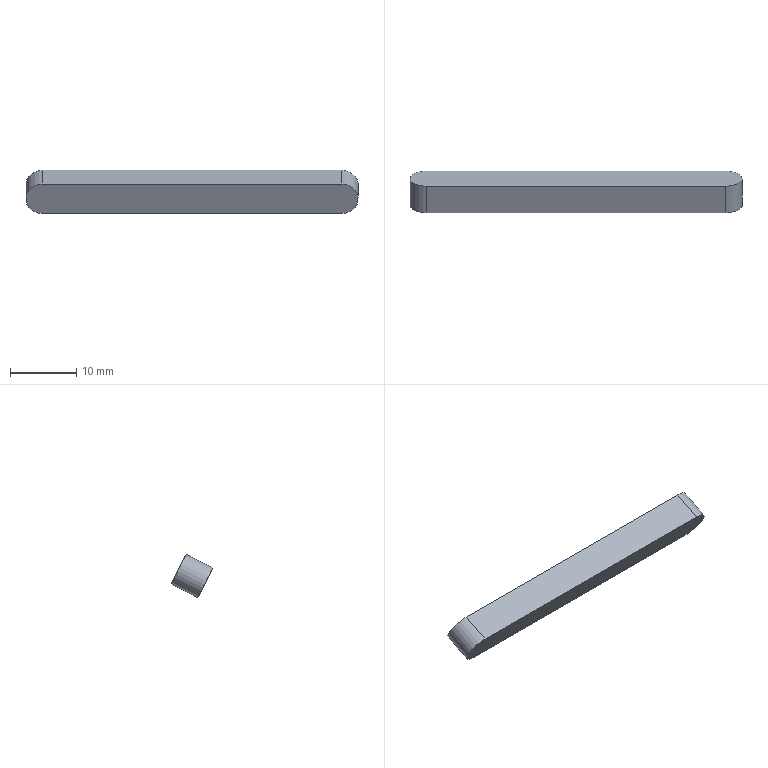Component | NX | KEY | 1 solid | 6 faces | box 50 x 6.28 x 6.5 mm | volume 1101 mm3 | plane 4 | cylinder 2 | commonest cylinder face diameters 5 x2
STEP:
#1=CARTESIAN_POINT('',(0.,0.,0.));
#2=DIRECTION('',(0.,0.,1.));
#3=DIRECTION('',(1.,0.,0.));
#4=AXIS2_PLACEMENT_3D('',#1,#2,#3);
#5=CARTESIAN_POINT('',(48.5,6.481,123.503));
#6=VERTEX_POINT('',#5);
#7=CARTESIAN_POINT('',(48.5,4.206,127.956));
#8=VERTEX_POINT('',#7);
#9=CARTESIAN_POINT('',(48.5,5.343,125.729));
#10=DIRECTION('',(0.,0.8906,0.4549));
#11=DIRECTION('',(1.,0.,0.));
#12=AXIS2_PLACEMENT_3D('',#9,#10,#11);
#13=CIRCLE('',#12,2.5);
#14=CARTESIAN_POINT('',(48.5,9.351,127.776));
#15=DIRECTION('',(0.,-0.8906,-0.4549));
#16=DIRECTION('',(-1.,0.,0.));
#17=AXIS2_PLACEMENT_3D('',#14,#15,#16);
#18=CYLINDRICAL_SURFACE('',#17,2.5);
#19=CARTESIAN_POINT('',(3.142,4.5));
#20=DIRECTION('',(-1.,-0.));
#21=VECTOR('',#20,1.);
#22=LINE('',#19,#21);
#23=(GEOMETRIC_REPRESENTATION_CONTEXT(2)PARAMETRIC_REPRESENTATION_CONTEXT()REPRESENTATION_CONTEXT('',''));
#24=DEFINITIONAL_REPRESENTATION('',(#22),#23);
#25=PCURVE('',#18,#24);
#26=CARTESIAN_POINT('',(48.5,5.343,125.729));
#27=DIRECTION('',(0.,0.8906,0.4549));
#28=DIRECTION('',(1.,0.,0.));
#29=AXIS2_PLACEMENT_3D('',#26,#27,#28);
#30=PLANE('',#29);
#31=CARTESIAN_POINT('',(0.,0.));
#32=DIRECTION('',(1.,0.));
#33=AXIS2_PLACEMENT_2D('',#31,#32);
#34=CIRCLE('',#33,2.5);
#35=(GEOMETRIC_REPRESENTATION_CONTEXT(2)PARAMETRIC_REPRESENTATION_CONTEXT()REPRESENTATION_CONTEXT('',''));
#36=DEFINITIONAL_REPRESENTATION('',(#34),#35);
#37=PCURVE('',#30,#36);
#38=SURFACE_CURVE('',#13,(#25,#37),.PCURVE_S1.);
#39=EDGE_CURVE('',#6,#8,#38,.T.);
#40=ORIENTED_EDGE('',*,*,#39,.T.);
#41=CARTESIAN_POINT('',(48.5,8.214,130.003));
#42=VERTEX_POINT('',#41);
#43=CARTESIAN_POINT('',(48.5,8.214,130.003));
#44=DIRECTION('',(0.,-0.8906,-0.4549));
#45=VECTOR('',#44,1.);
#46=LINE('',#43,#45);
#47=CARTESIAN_POINT('',(-1.571,-0.));
#48=DIRECTION('',(0.,1.));
#49=VECTOR('',#48,1.);
#50=LINE('',#47,#49);
#51=(GEOMETRIC_REPRESENTATION_CONTEXT(2)PARAMETRIC_REPRESENTATION_CONTEXT()REPRESENTATION_CONTEXT('',''));
#52=DEFINITIONAL_REPRESENTATION('',(#50),#51);
#53=PCURVE('',#18,#52);
#54=CARTESIAN_POINT('',(48.5,8.214,130.003));
#55=DIRECTION('',(0.,0.4549,-0.8906));
#56=DIRECTION('',(0.,0.8906,0.4549));
#57=AXIS2_PLACEMENT_3D('',#54,#55,#56);
#58=PLANE('',#57);
#59=CARTESIAN_POINT('',(0.,0.));
#60=DIRECTION('',(-1.,0.));
#61=VECTOR('',#60,1.);
#62=LINE('',#59,#61);
#63=(GEOMETRIC_REPRESENTATION_CONTEXT(2)PARAMETRIC_REPRESENTATION_CONTEXT()REPRESENTATION_CONTEXT('',''));
#64=DEFINITIONAL_REPRESENTATION('',(#62),#63);
#65=PCURVE('',#58,#64);
#66=SURFACE_CURVE('',#46,(#53,#65),.PCURVE_S1.);
#67=EDGE_CURVE('',#42,#8,#66,.T.);
#68=ORIENTED_EDGE('',*,*,#67,.F.);
#69=CARTESIAN_POINT('',(48.5,10.488,125.55));
#70=VERTEX_POINT('',#69);
#71=CARTESIAN_POINT('',(48.5,9.351,127.776));
#72=DIRECTION('',(0.,0.8906,0.4549));
#73=DIRECTION('',(1.,0.,0.));
#74=AXIS2_PLACEMENT_3D('',#71,#72,#73);
#75=CIRCLE('',#74,2.5);
#76=CARTESIAN_POINT('',(3.142,0.));
#77=DIRECTION('',(-1.,-0.));
#78=VECTOR('',#77,1.);
#79=LINE('',#76,#78);
#80=(GEOMETRIC_REPRESENTATION_CONTEXT(2)PARAMETRIC_REPRESENTATION_CONTEXT()REPRESENTATION_CONTEXT('',''));
#81=DEFINITIONAL_REPRESENTATION('',(#79),#80);
#82=PCURVE('',#18,#81);
#83=CARTESIAN_POINT('',(48.5,9.351,127.776));
#84=DIRECTION('',(0.,0.8906,0.4549));
#85=DIRECTION('',(1.,0.,0.));
#86=AXIS2_PLACEMENT_3D('',#83,#84,#85);
#87=PLANE('',#86);
#88=CARTESIAN_POINT('',(0.,0.));
#89=DIRECTION('',(1.,0.));
#90=AXIS2_PLACEMENT_2D('',#88,#89);
#91=CIRCLE('',#90,2.5);
#92=(GEOMETRIC_REPRESENTATION_CONTEXT(2)PARAMETRIC_REPRESENTATION_CONTEXT()REPRESENTATION_CONTEXT('',''));
#93=DEFINITIONAL_REPRESENTATION('',(#91),#92);
#94=PCURVE('',#87,#93);
#95=SURFACE_CURVE('',#75,(#82,#94),.PCURVE_S1.);
#96=EDGE_CURVE('',#70,#42,#95,.T.);
#97=ORIENTED_EDGE('',*,*,#96,.F.);
#98=CARTESIAN_POINT('',(48.5,10.488,125.55));
#99=DIRECTION('',(0.,-0.8906,-0.4549));
#100=VECTOR('',#99,1.);
#101=LINE('',#98,#100);
#102=CARTESIAN_POINT('',(1.571,0.));
#103=DIRECTION('',(0.,1.));
#104=VECTOR('',#103,1.);
#105=LINE('',#102,#104);
#106=(GEOMETRIC_REPRESENTATION_CONTEXT(2)PARAMETRIC_REPRESENTATION_CONTEXT()REPRESENTATION_CONTEXT('',''));
#107=DEFINITIONAL_REPRESENTATION('',(#105),#106);
#108=PCURVE('',#18,#107);
#109=CARTESIAN_POINT('',(93.5,10.488,125.55));
#110=DIRECTION('',(0.,-0.4549,0.8906));
#111=DIRECTION('',(0.,-0.8906,-0.4549));
#112=AXIS2_PLACEMENT_3D('',#109,#110,#111);
#113=PLANE('',#112);
#114=CARTESIAN_POINT('',(0.,-45.));
#115=DIRECTION('',(1.,0.));
#116=VECTOR('',#115,1.);
#117=LINE('',#114,#116);
#118=(GEOMETRIC_REPRESENTATION_CONTEXT(2)PARAMETRIC_REPRESENTATION_CONTEXT()REPRESENTATION_CONTEXT('',''));
#119=DEFINITIONAL_REPRESENTATION('',(#117),#118);
#120=PCURVE('',#113,#119);
#121=SURFACE_CURVE('',#101,(#108,#120),.PCURVE_S1.);
#122=EDGE_CURVE('',#70,#6,#121,.T.);
#123=ORIENTED_EDGE('',*,*,#122,.T.);
#124=EDGE_LOOP('',(#40,#68,#97,#123));
#125=FACE_BOUND('',#124,.T.);
#126=ADVANCED_FACE('',(#125),#18,.T.);
#127=CARTESIAN_POINT('',(93.5,4.206,127.956));
#128=VERTEX_POINT('',#127);
#129=CARTESIAN_POINT('',(48.5,4.206,127.956));
#130=DIRECTION('',(1.,0.,0.));
#131=VECTOR('',#130,1.);
#132=LINE('',#129,#131);
#133=CARTESIAN_POINT('',(-4.5,0.));
#134=DIRECTION('',(0.,1.));
#135=VECTOR('',#134,1.);
#136=LINE('',#133,#135);
#137=(GEOMETRIC_REPRESENTATION_CONTEXT(2)PARAMETRIC_REPRESENTATION_CONTEXT()REPRESENTATION_CONTEXT('',''));
#138=DEFINITIONAL_REPRESENTATION('',(#136),#137);
#139=PCURVE('',#58,#138);
#140=CARTESIAN_POINT('',(0.,-2.5));
#141=DIRECTION('',(1.,0.));
#142=VECTOR('',#141,1.);
#143=LINE('',#140,#142);
#144=(GEOMETRIC_REPRESENTATION_CONTEXT(2)PARAMETRIC_REPRESENTATION_CONTEXT()REPRESENTATION_CONTEXT('',''));
#145=DEFINITIONAL_REPRESENTATION('',(#143),#144);
#146=PCURVE('',#30,#145);
#147=SURFACE_CURVE('',#132,(#139,#146),.PCURVE_S1.);
#148=EDGE_CURVE('',#8,#128,#147,.T.);
#149=ORIENTED_EDGE('',*,*,#148,.T.);
#150=CARTESIAN_POINT('',(93.5,8.214,130.003));
#151=VERTEX_POINT('',#150);
#152=CARTESIAN_POINT('',(93.5,8.214,130.003));
#153=DIRECTION('',(0.,-0.8906,-0.4549));
#154=VECTOR('',#153,1.);
#155=LINE('',#152,#154);
#156=CARTESIAN_POINT('',(0.,45.));
#157=DIRECTION('',(-1.,0.));
#158=VECTOR('',#157,1.);
#159=LINE('',#156,#158);
#160=(GEOMETRIC_REPRESENTATION_CONTEXT(2)PARAMETRIC_REPRESENTATION_CONTEXT()REPRESENTATION_CONTEXT('',''));
#161=DEFINITIONAL_REPRESENTATION('',(#159),#160);
#162=PCURVE('',#58,#161);
#163=CARTESIAN_POINT('',(93.5,9.351,127.776));
#164=DIRECTION('',(0.,-0.8906,-0.4549));
#165=DIRECTION('',(-1.,0.,0.));
#166=AXIS2_PLACEMENT_3D('',#163,#164,#165);
#167=CYLINDRICAL_SURFACE('',#166,2.5);
#168=CARTESIAN_POINT('',(4.712,-0.));
#169=DIRECTION('',(0.,1.));
#170=VECTOR('',#169,1.);
#171=LINE('',#168,#170);
#172=(GEOMETRIC_REPRESENTATION_CONTEXT(2)PARAMETRIC_REPRESENTATION_CONTEXT()REPRESENTATION_CONTEXT('',''));
#173=DEFINITIONAL_REPRESENTATION('',(#171),#172);
#174=PCURVE('',#167,#173);
#175=SURFACE_CURVE('',#155,(#162,#174),.PCURVE_S1.);
#176=EDGE_CURVE('',#151,#128,#175,.T.);
#177=ORIENTED_EDGE('',*,*,#176,.F.);
#178=CARTESIAN_POINT('',(48.5,8.214,130.003));
#179=DIRECTION('',(1.,0.,0.));
#180=VECTOR('',#179,1.);
#181=LINE('',#178,#180);
#182=CARTESIAN_POINT('',(0.,0.));
#183=DIRECTION('',(0.,1.));
#184=VECTOR('',#183,1.);
#185=LINE('',#182,#184);
#186=(GEOMETRIC_REPRESENTATION_CONTEXT(2)PARAMETRIC_REPRESENTATION_CONTEXT()REPRESENTATION_CONTEXT('',''));
#187=DEFINITIONAL_REPRESENTATION('',(#185),#186);
#188=PCURVE('',#58,#187);
#189=CARTESIAN_POINT('',(0.,-2.5));
#190=DIRECTION('',(1.,0.));
#191=VECTOR('',#190,1.);
#192=LINE('',#189,#191);
#193=(GEOMETRIC_REPRESENTATION_CONTEXT(2)PARAMETRIC_REPRESENTATION_CONTEXT()REPRESENTATION_CONTEXT('',''));
#194=DEFINITIONAL_REPRESENTATION('',(#192),#193);
#195=PCURVE('',#87,#194);
#196=SURFACE_CURVE('',#181,(#188,#195),.PCURVE_S1.);
#197=EDGE_CURVE('',#42,#151,#196,.T.);
#198=ORIENTED_EDGE('',*,*,#197,.F.);
#199=ORIENTED_EDGE('',*,*,#67,.T.);
#200=EDGE_LOOP('',(#149,#177,#198,#199));
#201=FACE_BOUND('',#200,.T.);
#202=ADVANCED_FACE('',(#201),#58,.F.);
#203=CARTESIAN_POINT('',(93.5,6.481,123.503));
#204=VERTEX_POINT('',#203);
#205=CARTESIAN_POINT('',(93.5,5.343,125.729));
#206=DIRECTION('',(0.,0.8906,0.4549));
#207=DIRECTION('',(-1.,0.,0.));
#208=AXIS2_PLACEMENT_3D('',#205,#206,#207);
#209=CIRCLE('',#208,2.5);
#210=CARTESIAN_POINT('',(6.283,4.5));
#211=DIRECTION('',(-1.,0.));
#212=VECTOR('',#211,1.);
#213=LINE('',#210,#212);
#214=(GEOMETRIC_REPRESENTATION_CONTEXT(2)PARAMETRIC_REPRESENTATION_CONTEXT()REPRESENTATION_CONTEXT('',''));
#215=DEFINITIONAL_REPRESENTATION('',(#213),#214);
#216=PCURVE('',#167,#215);
#217=CARTESIAN_POINT('',(45.,0.));
#218=DIRECTION('',(-1.,0.));
#219=AXIS2_PLACEMENT_2D('',#217,#218);
#220=CIRCLE('',#219,2.5);
#221=(GEOMETRIC_REPRESENTATION_CONTEXT(2)PARAMETRIC_REPRESENTATION_CONTEXT()REPRESENTATION_CONTEXT('',''));
#222=DEFINITIONAL_REPRESENTATION('',(#220),#221);
#223=PCURVE('',#30,#222);
#224=SURFACE_CURVE('',#209,(#216,#223),.PCURVE_S1.);
#225=EDGE_CURVE('',#128,#204,#224,.T.);
#226=ORIENTED_EDGE('',*,*,#225,.T.);
#227=CARTESIAN_POINT('',(93.5,10.488,125.55));
#228=VERTEX_POINT('',#227);
#229=CARTESIAN_POINT('',(93.5,10.488,125.55));
#230=DIRECTION('',(0.,-0.8906,-0.4549));
#231=VECTOR('',#230,1.);
#232=LINE('',#229,#231);
#233=CARTESIAN_POINT('',(1.571,0.));
#234=DIRECTION('',(0.,1.));
#235=VECTOR('',#234,1.);
#236=LINE('',#233,#235);
#237=(GEOMETRIC_REPRESENTATION_CONTEXT(2)PARAMETRIC_REPRESENTATION_CONTEXT()REPRESENTATION_CONTEXT('',''));
#238=DEFINITIONAL_REPRESENTATION('',(#236),#237);
#239=PCURVE('',#167,#238);
#240=CARTESIAN_POINT('',(0.,-0.));
#241=DIRECTION('',(1.,0.));
#242=VECTOR('',#241,1.);
#243=LINE('',#240,#242);
#244=(GEOMETRIC_REPRESENTATION_CONTEXT(2)PARAMETRIC_REPRESENTATION_CONTEXT()REPRESENTATION_CONTEXT('',''));
#245=DEFINITIONAL_REPRESENTATION('',(#243),#244);
#246=PCURVE('',#113,#245);
#247=SURFACE_CURVE('',#232,(#239,#246),.PCURVE_S1.);
#248=EDGE_CURVE('',#228,#204,#247,.T.);
#249=ORIENTED_EDGE('',*,*,#248,.F.);
#250=CARTESIAN_POINT('',(93.5,9.351,127.776));
#251=DIRECTION('',(0.,0.8906,0.4549));
#252=DIRECTION('',(-1.,0.,0.));
#253=AXIS2_PLACEMENT_3D('',#250,#251,#252);
#254=CIRCLE('',#253,2.5);
#255=CARTESIAN_POINT('',(6.283,-0.));
#256=DIRECTION('',(-1.,0.));
#257=VECTOR('',#256,1.);
#258=LINE('',#255,#257);
#259=(GEOMETRIC_REPRESENTATION_CONTEXT(2)PARAMETRIC_REPRESENTATION_CONTEXT()REPRESENTATION_CONTEXT('',''));
#260=DEFINITIONAL_REPRESENTATION('',(#258),#259);
#261=PCURVE('',#167,#260);
#262=CARTESIAN_POINT('',(45.,0.));
#263=DIRECTION('',(-1.,0.));
#264=AXIS2_PLACEMENT_2D('',#262,#263);
#265=CIRCLE('',#264,2.5);
#266=(GEOMETRIC_REPRESENTATION_CONTEXT(2)PARAMETRIC_REPRESENTATION_CONTEXT()REPRESENTATION_CONTEXT('',''));
#267=DEFINITIONAL_REPRESENTATION('',(#265),#266);
#268=PCURVE('',#87,#267);
#269=SURFACE_CURVE('',#254,(#261,#268),.PCURVE_S1.);
#270=EDGE_CURVE('',#151,#228,#269,.T.);
#271=ORIENTED_EDGE('',*,*,#270,.F.);
#272=ORIENTED_EDGE('',*,*,#176,.T.);
#273=EDGE_LOOP('',(#226,#249,#271,#272));
#274=FACE_BOUND('',#273,.T.);
#275=ADVANCED_FACE('',(#274),#167,.T.);
#276=CARTESIAN_POINT('',(93.5,6.481,123.503));
#277=DIRECTION('',(-1.,0.,0.));
#278=VECTOR('',#277,1.);
#279=LINE('',#276,#278);
#280=CARTESIAN_POINT('',(4.5,0.));
#281=DIRECTION('',(0.,-1.));
#282=VECTOR('',#281,1.);
#283=LINE('',#280,#282);
#284=(GEOMETRIC_REPRESENTATION_CONTEXT(2)PARAMETRIC_REPRESENTATION_CONTEXT()REPRESENTATION_CONTEXT('',''));
#285=DEFINITIONAL_REPRESENTATION('',(#283),#284);
#286=PCURVE('',#113,#285);
#287=CARTESIAN_POINT('',(45.,2.5));
#288=DIRECTION('',(-1.,0.));
#289=VECTOR('',#288,1.);
#290=LINE('',#287,#289);
#291=(GEOMETRIC_REPRESENTATION_CONTEXT(2)PARAMETRIC_REPRESENTATION_CONTEXT()REPRESENTATION_CONTEXT('',''));
#292=DEFINITIONAL_REPRESENTATION('',(#290),#291);
#293=PCURVE('',#30,#292);
#294=SURFACE_CURVE('',#279,(#286,#293),.PCURVE_S1.);
#295=EDGE_CURVE('',#204,#6,#294,.T.);
#296=ORIENTED_EDGE('',*,*,#295,.T.);
#297=ORIENTED_EDGE('',*,*,#122,.F.);
#298=CARTESIAN_POINT('',(93.5,10.488,125.55));
#299=DIRECTION('',(-1.,0.,0.));
#300=VECTOR('',#299,1.);
#301=LINE('',#298,#300);
#302=CARTESIAN_POINT('',(0.,0.));
#303=DIRECTION('',(0.,-1.));
#304=VECTOR('',#303,1.);
#305=LINE('',#302,#304);
#306=(GEOMETRIC_REPRESENTATION_CONTEXT(2)PARAMETRIC_REPRESENTATION_CONTEXT()REPRESENTATION_CONTEXT('',''));
#307=DEFINITIONAL_REPRESENTATION('',(#305),#306);
#308=PCURVE('',#113,#307);
#309=CARTESIAN_POINT('',(45.,2.5));
#310=DIRECTION('',(-1.,0.));
#311=VECTOR('',#310,1.);
#312=LINE('',#309,#311);
#313=(GEOMETRIC_REPRESENTATION_CONTEXT(2)PARAMETRIC_REPRESENTATION_CONTEXT()REPRESENTATION_CONTEXT('',''));
#314=DEFINITIONAL_REPRESENTATION('',(#312),#313);
#315=PCURVE('',#87,#314);
#316=SURFACE_CURVE('',#301,(#308,#315),.PCURVE_S1.);
#317=EDGE_CURVE('',#228,#70,#316,.T.);
#318=ORIENTED_EDGE('',*,*,#317,.F.);
#319=ORIENTED_EDGE('',*,*,#248,.T.);
#320=EDGE_LOOP('',(#296,#297,#318,#319));
#321=FACE_BOUND('',#320,.T.);
#322=ADVANCED_FACE('',(#321),#113,.F.);
#323=ORIENTED_EDGE('',*,*,#96,.T.);
#324=ORIENTED_EDGE('',*,*,#197,.T.);
#325=ORIENTED_EDGE('',*,*,#270,.T.);
#326=ORIENTED_EDGE('',*,*,#317,.T.);
#327=EDGE_LOOP('',(#323,#324,#325,#326));
#328=FACE_BOUND('',#327,.T.);
#329=ADVANCED_FACE('',(#328),#87,.T.);
#330=ORIENTED_EDGE('',*,*,#39,.F.);
#331=ORIENTED_EDGE('',*,*,#295,.F.);
#332=ORIENTED_EDGE('',*,*,#225,.F.);
#333=ORIENTED_EDGE('',*,*,#148,.F.);
#334=EDGE_LOOP('',(#330,#331,#332,#333));
#335=FACE_BOUND('',#334,.T.);
#336=ADVANCED_FACE('',(#335),#30,.F.);
#337=CLOSED_SHELL('',(#126,#202,#275,#322,#329,#336));
#338=MANIFOLD_SOLID_BREP('',#337);
#339=(LENGTH_UNIT()NAMED_UNIT(*)SI_UNIT(.MILLI.,.METRE.));
#340=UNCERTAINTY_MEASURE_WITH_UNIT(LENGTH_MEASURE(0.0000001),#339,'','');
#341=(NAMED_UNIT(*)PLANE_ANGLE_UNIT()SI_UNIT($,.RADIAN.));
#342=(NAMED_UNIT(*)SI_UNIT($,.STERADIAN.)SOLID_ANGLE_UNIT());
#343=(GEOMETRIC_REPRESENTATION_CONTEXT(3)GLOBAL_UNCERTAINTY_ASSIGNED_CONTEXT((#340))GLOBAL_UNIT_ASSIGNED_CONTEXT((#339,#341,#342))REPRESENTATION_CONTEXT('',''));
#344=ADVANCED_BREP_SHAPE_REPRESENTATION('',(#4,#338),#343);